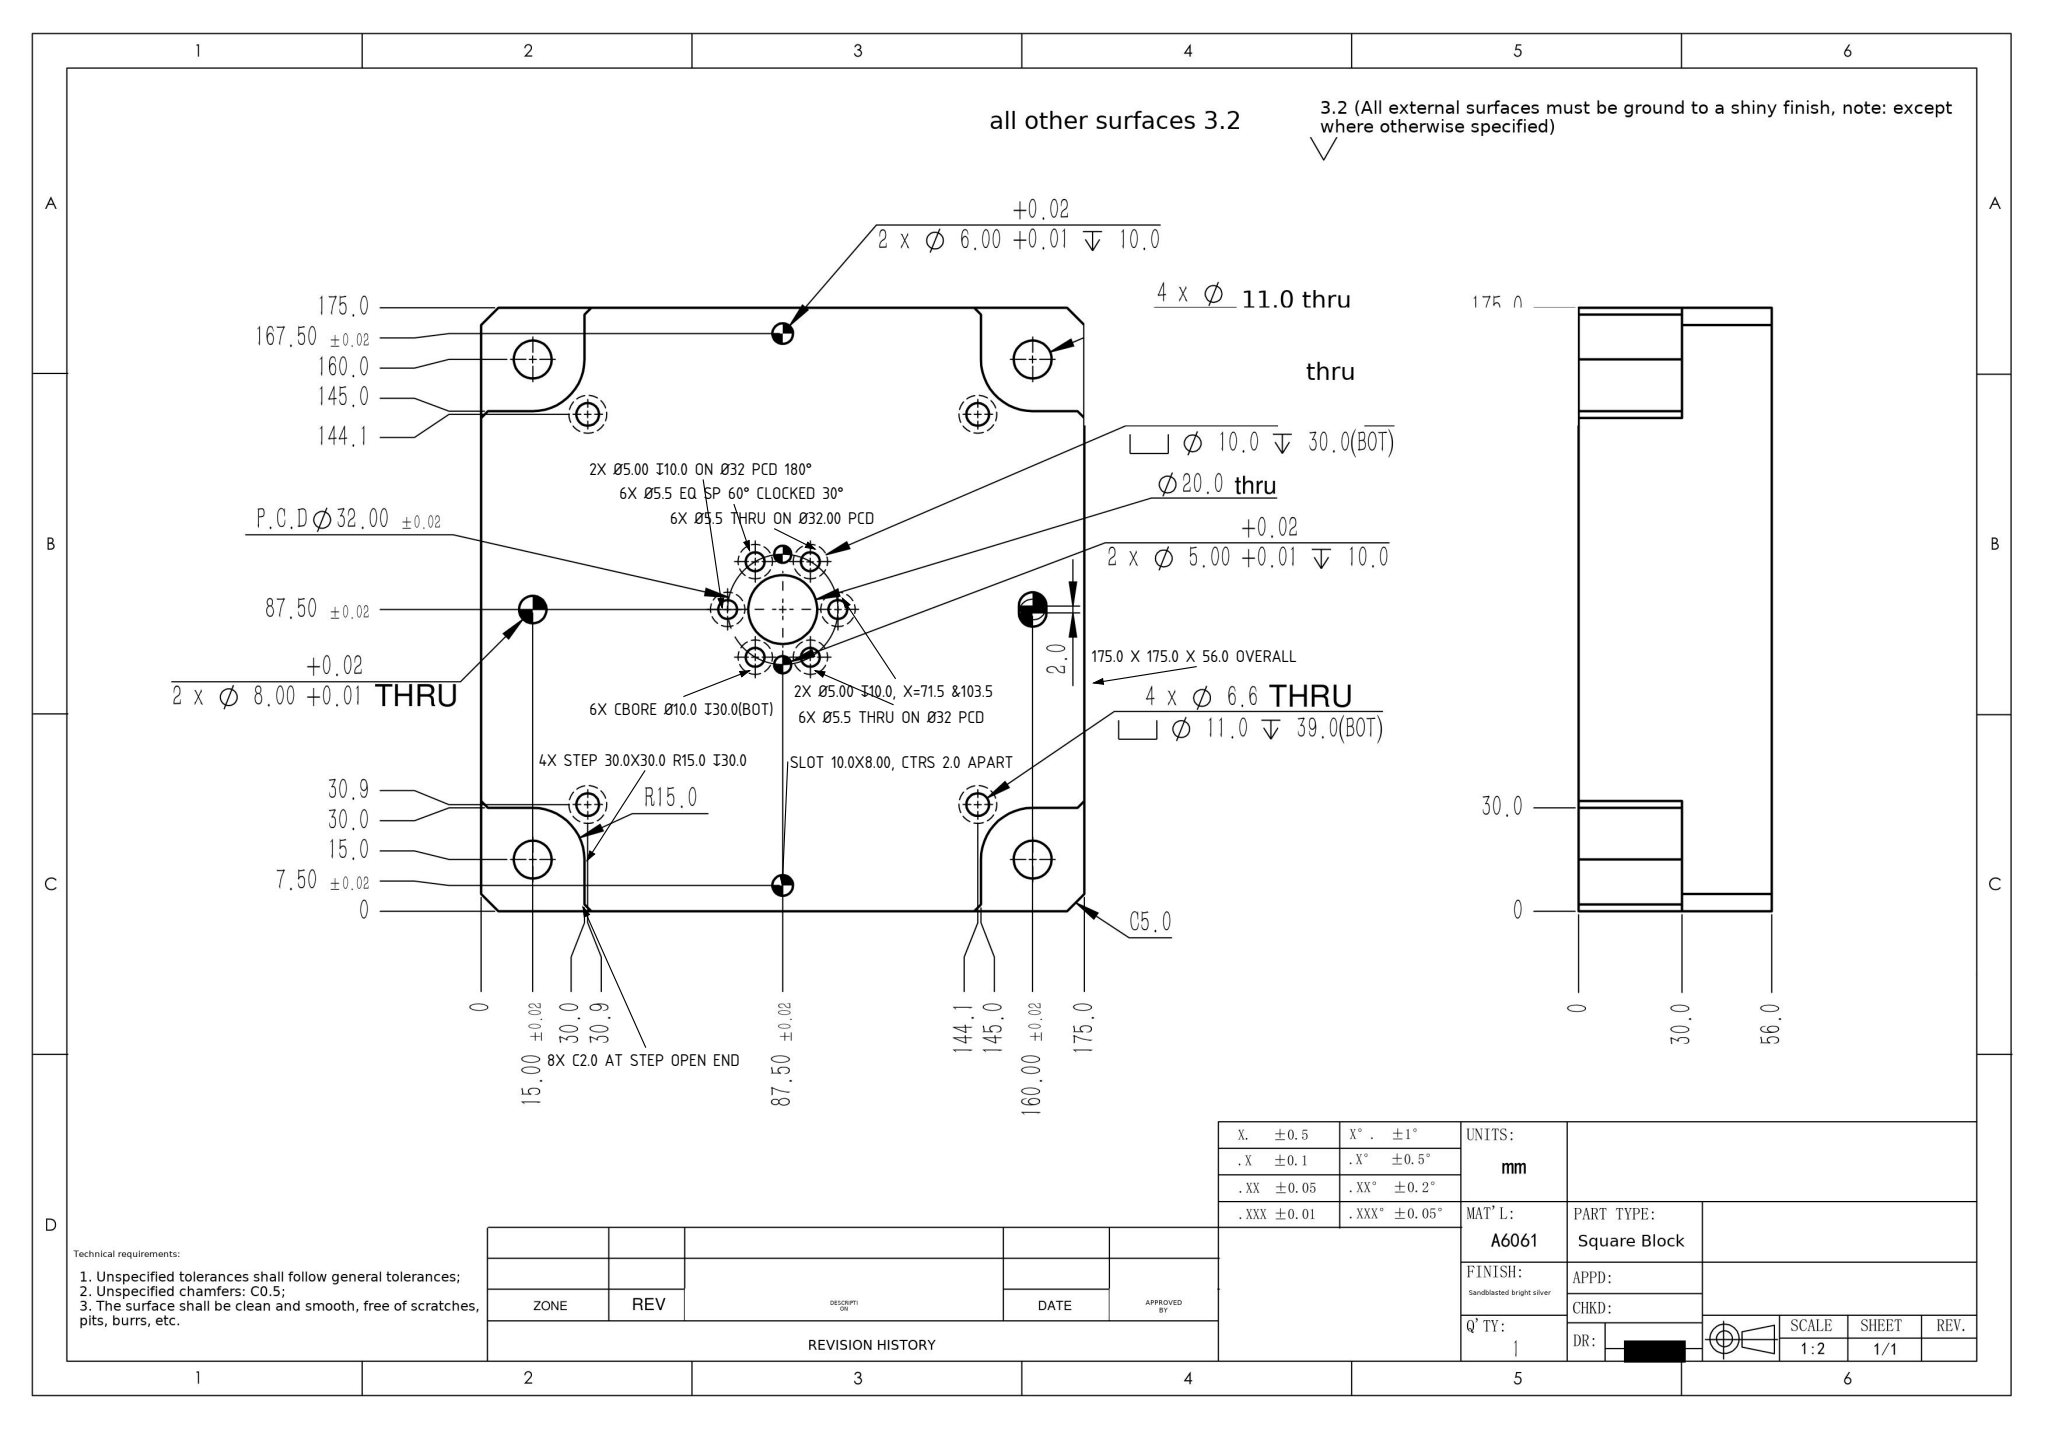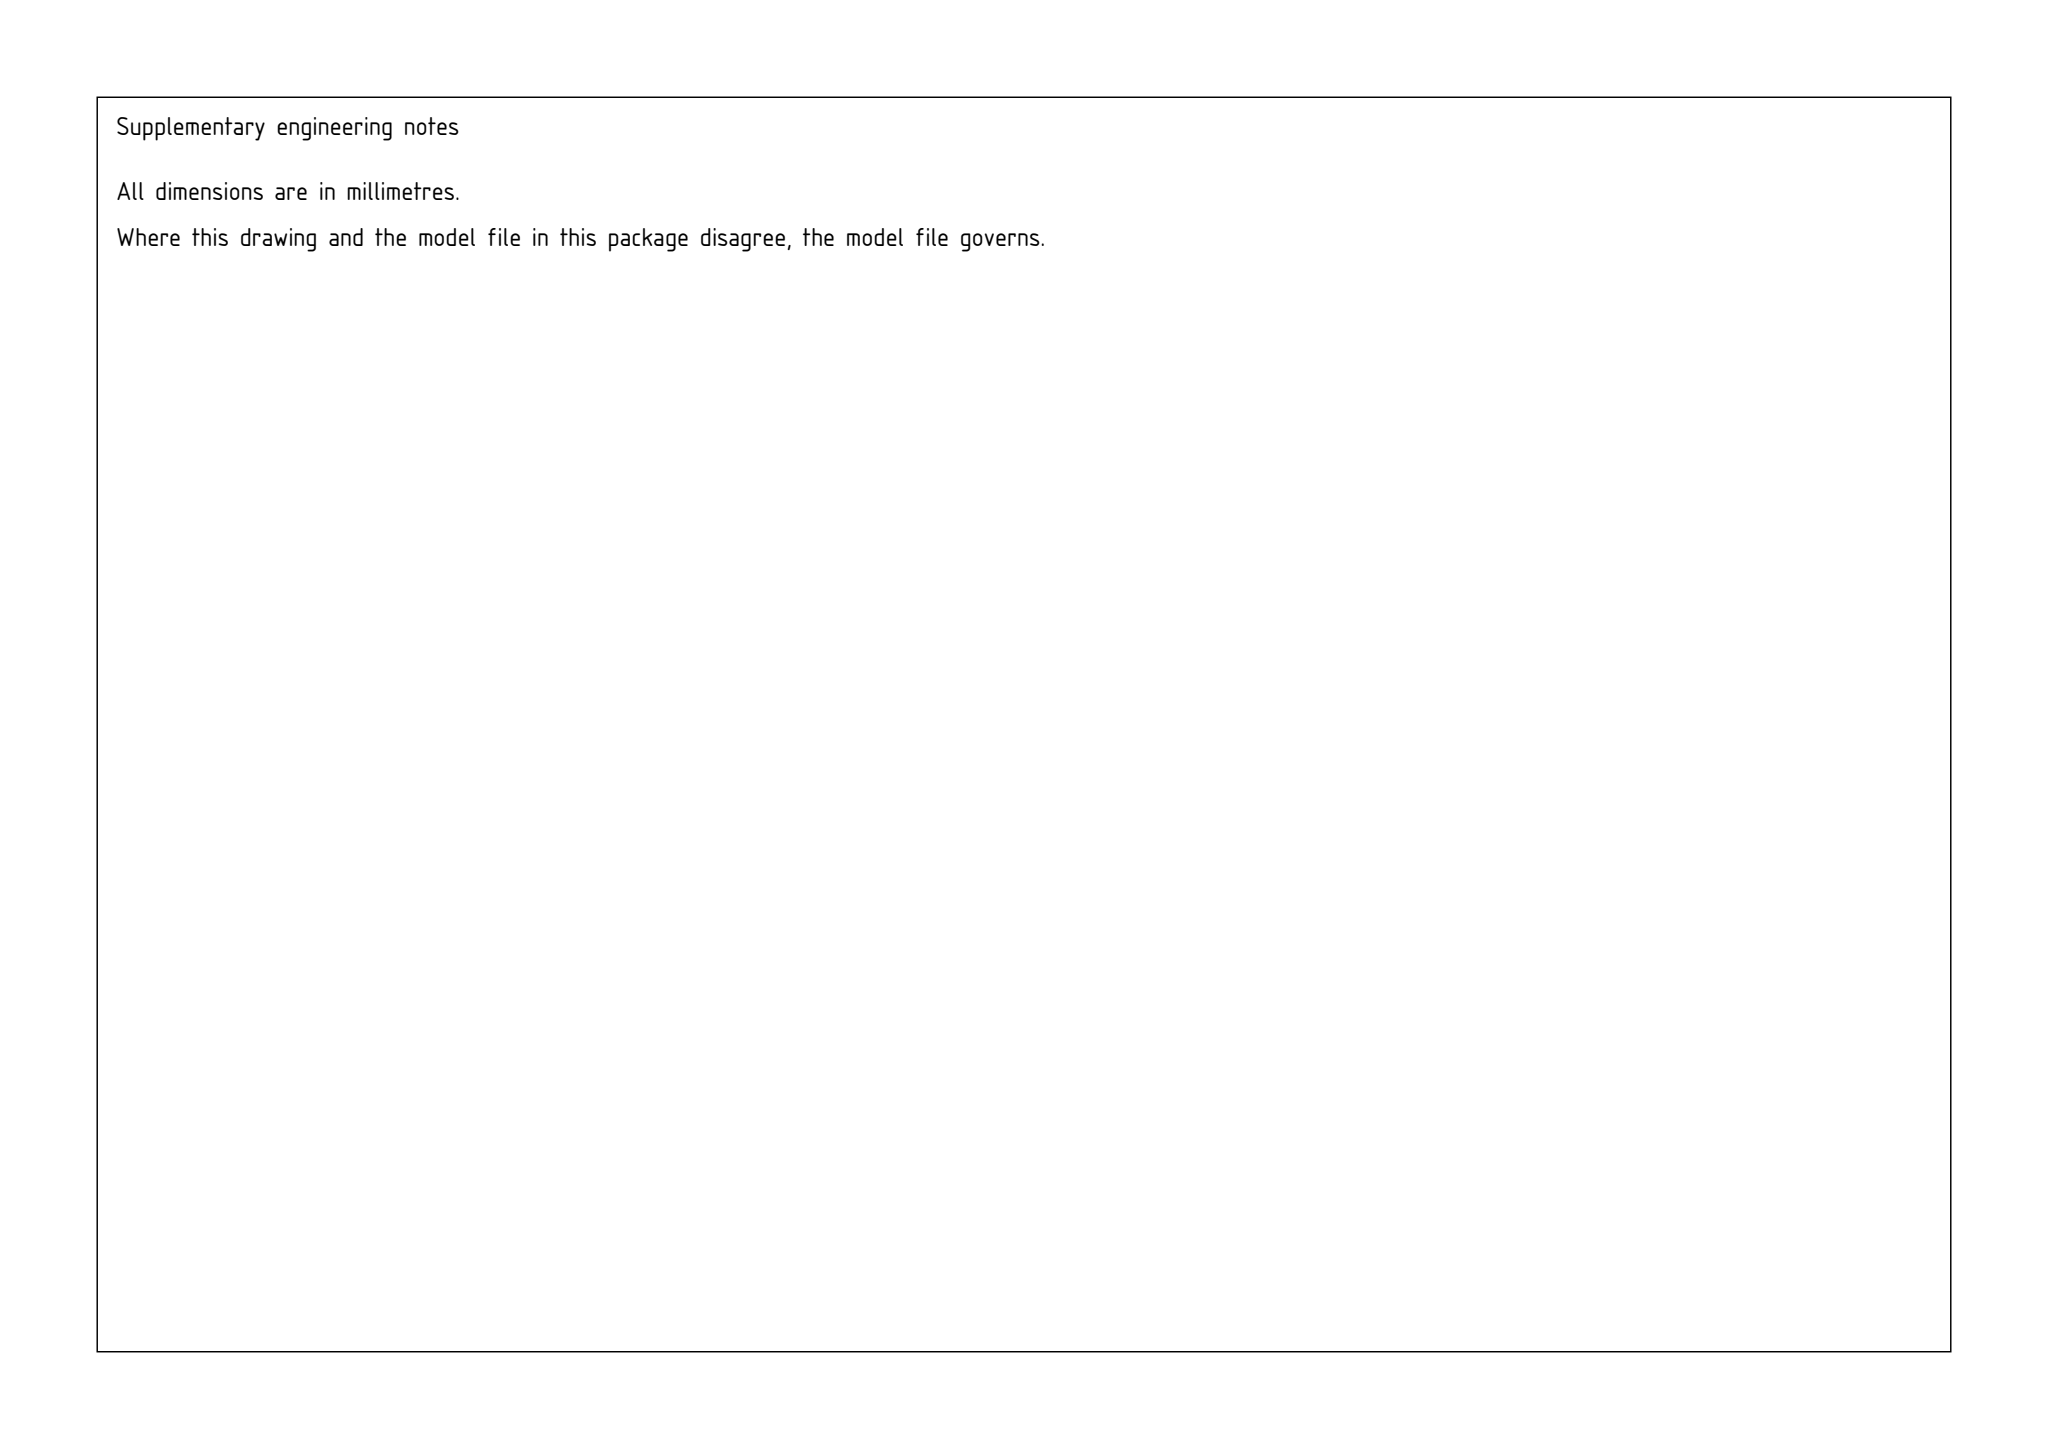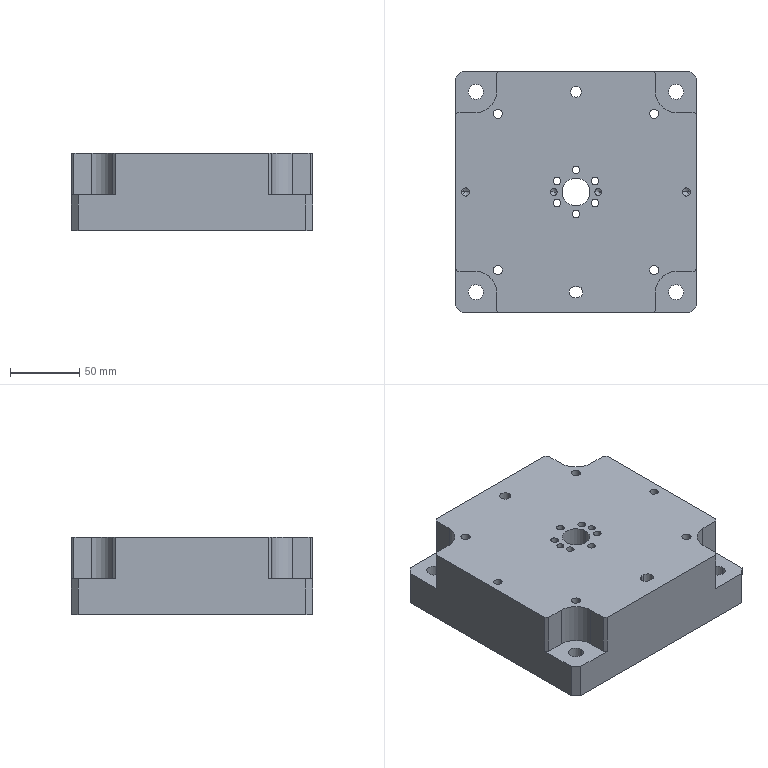Part | SolidWorks | mm | material A6061 | 1 solid | 117 faces | box 175 x 175 x 56 mm | volume 1541005 mm3 | cylinder 67 | plane 42 | cone 8 | commonest cylinder face diameters 11 x16 10 x12 5.5 x12 6.6 x8 8 x5 5 x4 6 x4 30 x4
Drawing notes:
OVERALL 175.0 X 175.0 X 56.0 | from the solid: bbox_xyz [175.0, 175.0, 56.0]
4 X CORNER STEP 30.0 X 30.0, R15.0, DP 30.0 FROM TOP, FLOOR Z=26.0 | from the solid: x & y planes at 30.0 and 145.0 (2 ea); 4 x z=26.0 faces; R15 (Ø30) fillet cyl len 30 at (15,15),(15,160),(160,15),(160,160)
6 X Ø5.5 THRU ON Ø32.00 PCD, 1ST 30° FROM HORIZ SP 60°, CTR 87.50,87.50 | from the solid: Ø5.5 holes at (73.64,79.5),(73.64,95.5),(87.5,71.5),(87.5,103.5),(101.36,79.5),(101.36,95.5) = R16.0 at 30/90/150/210/270/330° about (87.5,87.5), len 26 to z=56
CBORE Ø10.0 DP 30.0(BOT) ALL 6 PCD HOLES | from the solid: 6 x Ø10.0 cyl len 30 from z=0 at PCD positions; 6 x z=30.0 cbore floors
2 X Ø5.00 DP 10.0 ON CL Y=87.50, X=71.50 & 103.50, 16.0 EA SIDE OF Ø20 | from the solid: Ø5.0 z-axis holes at (71.5,87.5) and (103.5,87.5), length 10.0; Ø20 thru at (87.5,87.5)
Ø8.00 THRU AT Y=15.0 SLOTTED: 10.0 O/A X 8.00 WIDE, CTRS 2.0 APART | from the solid: Ø8.0 thru cyls at x=86.5 and x=88.5, y=15.0, len 56; flats y=11.0 & y=19.0
6X Ø5.5 ON Ø32 PCD, EQ SP 60°, CLOCKED 30° FROM HORIZ CL | from the solid: Ø5.5 holes at (101.4,79.5),(101.4,95.5),(73.6,79.5),(73.6,95.5),(87.5,103.5),(87.5,71.5) about ctr 87.5,87.5 = R16 at -30/30/210/150/90/270 deg
2X Ø5.00 DP 10.0 ON Ø32 PCD AT 0° & 180°, ON HORIZ CL | from the solid: Ø5.0 holes at (103.5,87.5) and (71.5,87.5), R16 from ctr 87.5,87.5, z 46-56 (10 deep from top)
CORNER STEP 30.0 WIDE x 30.0 DP, C2 AT OPEN END, 8 PLCS | from the solid: 45° planes size 2x2x30 at z26-56 (x/y 30,143,173...); step faces x=30/145, y=30/145, z=26 pads 32x32 → 30.0 wide, opening 32.0
6X Ø5.5 ON Ø32 PCD EQ SP 60°, CLOCKED 30° FROM HORIZ C/L | from the solid: Ø5.5 holes at (101.4,79.5),(101.4,95.5),(73.6,79.5),(73.6,95.5),(87.5,103.5),(87.5,71.5) about center (87.5,87.5); r=16 => 30/90/150/210/270/330°, vs 2X Ø5.00 at (103.5,87.5)&(71.5,87.5) = 0/180°